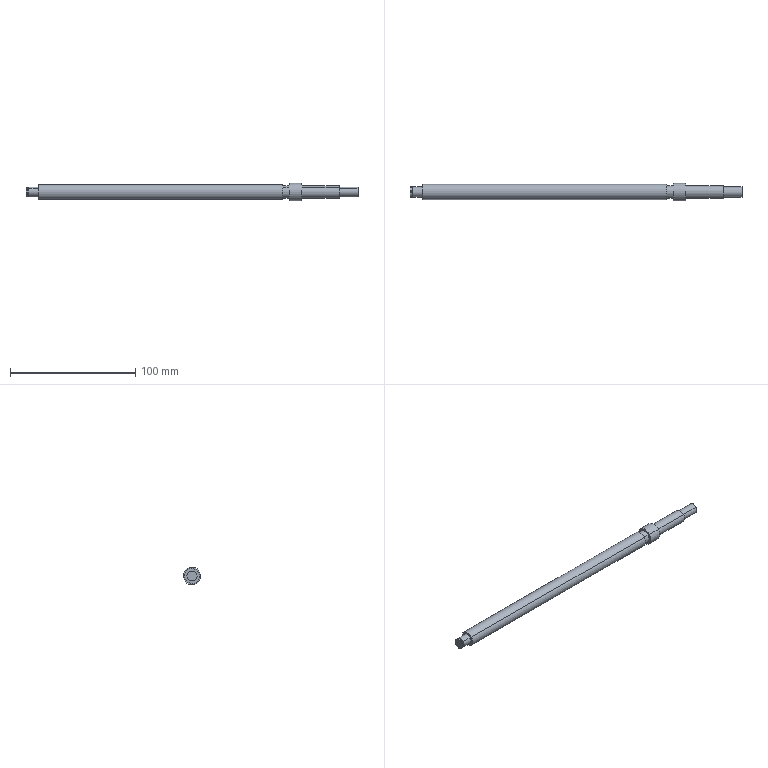Component | SolidWorks | BNK1208-2-ScrewRod-1 | 1 solid | 25 faces | box 265 x 14 x 14 mm | volume 27592 mm3 | cylinder 16 | plane 9 | commonest cylinder face diameters 8 x6 10 x4 7.4 x2 12 x2 14 x2
build123d program:
from build123d import *

# Parameters (mm, degrees)
SKETCH1_R           = 4
BOSS_EXTRUDE1_DEPTH = 15
SKETCH2_R           = 5
BOSS_EXTRUDE2_DEPTH = 30
SKETCH3_R           = 7
BOSS_EXTRUDE3_DEPTH = 10
SKETCH4_R           = 5
BOSS_EXTRUDE4_DEPTH = 5
SKETCH5_R           = 6
BOSS_EXTRUDE5_DEPTH = 195
SKETCH6_R           = 4
BOSS_EXTRUDE6_DEPTH = 10
SKETCH7_W           = 0.3
SKETCH7_H           = 0.9


with BuildPart() as part:
    # Sketch1 → Boss-Extrude1 (new body)
    with BuildSketch(Plane.XY):
        Circle(SKETCH1_R)
    extrude(amount=BOSS_EXTRUDE1_DEPTH)

    # Sketch2 → Boss-Extrude2 (add)
    with BuildSketch(Plane.XY.offset(15)):
        Circle(SKETCH2_R)
    extrude(amount=BOSS_EXTRUDE2_DEPTH)

    # Sketch3 → Boss-Extrude3 (add)
    with BuildSketch(Plane.XY.offset(45)):
        Circle(SKETCH3_R)
    extrude(amount=BOSS_EXTRUDE3_DEPTH)

    # Sketch4 → Boss-Extrude4 (add)
    with BuildSketch(Plane.XY.offset(55)):
        Circle(SKETCH4_R)
    extrude(amount=BOSS_EXTRUDE4_DEPTH)

    # Sketch5 → Boss-Extrude5 (add)
    with BuildSketch(Plane.XY.offset(60)):
        Circle(SKETCH5_R)
    extrude(amount=BOSS_EXTRUDE5_DEPTH)

    # Sketch6 → Boss-Extrude6 (add)
    with BuildSketch(Plane.XY.offset(255)):
        Circle(SKETCH6_R)
    extrude(amount=BOSS_EXTRUDE6_DEPTH)

    # Sketch7 → Cut-Revolve1 (revolve, cut)
    with BuildSketch(Plane(origin=(0, 0, 0), x_dir=(1, 0, 0), z_dir=(0, 1, 0)), mode=Mode.PRIVATE) as cut_revolve1_sk:
        with Locations((-3.85, -263.35)):
            Rectangle(SKETCH7_W, SKETCH7_H)
    revolve(cut_revolve1_sk.sketch.rotate(Axis((0, 0, 255), (0, 0, -1)), 180), axis=Axis((0, 0, 255), (0, 0, -1)), mode=Mode.SUBTRACT)


solid = part.part

# Placed as in the assembly
solid = solid.moved(Location((73.978, 19.945, 3.551), (0, -90, 0)))
STEP:
#1=CARTESIAN_POINT('',(-7.521,0.9056,0.03818));
#2=VERTEX_POINT('',#1);
#3=CARTESIAN_POINT('',(-7.521,0.6649,0.2414));
#4=VERTEX_POINT('',#3);
#5=CARTESIAN_POINT('',(-7.521,0.7853,0.1398));
#6=DIRECTION('',(-1.,0.,0.));
#7=DIRECTION('',(0.,0.764,-0.6453));
#8=AXIS2_PLACEMENT_3D('',#5,#6,#7);
#9=CIRCLE('',#8,0.1575);
#10=EDGE_CURVE('',#2,#4,#9,.T.);
#11=ORIENTED_EDGE('',*,*,#10,.F.);
#12=CARTESIAN_POINT('',(-7.473,0.9056,0.03818));
#13=VERTEX_POINT('',#12);
#14=CARTESIAN_POINT('',(-7.521,0.9056,0.03818));
#15=DIRECTION('',(1.,-0.,-0.));
#16=VECTOR('',#15,39.37);
#17=LINE('',#14,#16);
#18=EDGE_CURVE('',#2,#13,#17,.T.);
#19=ORIENTED_EDGE('',*,*,#18,.T.);
#20=CARTESIAN_POINT('',(-7.473,0.6649,0.2414));
#21=VERTEX_POINT('',#20);
#22=CARTESIAN_POINT('',(-7.473,0.7853,0.1398));
#23=DIRECTION('',(-1.,0.,0.));
#24=DIRECTION('',(0.,0.764,-0.6453));
#25=AXIS2_PLACEMENT_3D('',#22,#23,#24);
#26=CIRCLE('',#25,0.1575);
#27=EDGE_CURVE('',#13,#21,#26,.T.);
#28=ORIENTED_EDGE('',*,*,#27,.T.);
#29=CARTESIAN_POINT('',(-7.521,0.6649,0.2414));
#30=DIRECTION('',(1.,-0.,-0.));
#31=VECTOR('',#30,39.37);
#32=LINE('',#29,#31);
#33=EDGE_CURVE('',#4,#21,#32,.T.);
#34=ORIENTED_EDGE('',*,*,#33,.F.);
#35=EDGE_LOOP('',(#11,#19,#28,#34));
#36=FACE_OUTER_BOUND('',#35,.T.);
#37=CARTESIAN_POINT('',(-7.521,0.7853,0.1398));
#38=DIRECTION('',(1.,-0.,-0.));
#39=DIRECTION('',(0.,-0.764,0.6453));
#40=AXIS2_PLACEMENT_3D('',#37,#38,#39);
#41=CYLINDRICAL_SURFACE('',#40,0.1575);
#42=ADVANCED_FACE('',(#36),#41,.T.);
#43=CARTESIAN_POINT('',(-7.438,0.8965,0.0458));
#44=VERTEX_POINT('',#43);
#45=CARTESIAN_POINT('',(-7.438,0.674,0.2338));
#46=VERTEX_POINT('',#45);
#47=CARTESIAN_POINT('',(-7.438,0.7853,0.1398));
#48=DIRECTION('',(-1.,0.,0.));
#49=DIRECTION('',(0.,0.764,-0.6453));
#50=AXIS2_PLACEMENT_3D('',#47,#48,#49);
#51=CIRCLE('',#50,0.1457);
#52=EDGE_CURVE('',#44,#46,#51,.T.);
#53=ORIENTED_EDGE('',*,*,#52,.T.);
#54=CARTESIAN_POINT('',(-7.473,0.674,0.2338));
#55=VERTEX_POINT('',#54);
#56=CARTESIAN_POINT('',(-7.127,0.674,0.2338));
#57=DIRECTION('',(-1.,0.,0.));
#58=VECTOR('',#57,39.37);
#59=LINE('',#56,#58);
#60=EDGE_CURVE('',#46,#55,#59,.T.);
#61=ORIENTED_EDGE('',*,*,#60,.T.);
#62=CARTESIAN_POINT('',(-7.473,0.8965,0.0458));
#63=VERTEX_POINT('',#62);
#64=CARTESIAN_POINT('',(-7.473,0.7853,0.1398));
#65=DIRECTION('',(-1.,0.,0.));
#66=DIRECTION('',(0.,0.764,-0.6453));
#67=AXIS2_PLACEMENT_3D('',#64,#65,#66);
#68=CIRCLE('',#67,0.1457);
#69=EDGE_CURVE('',#63,#55,#68,.T.);
#70=ORIENTED_EDGE('',*,*,#69,.F.);
#71=CARTESIAN_POINT('',(-7.127,0.8965,0.0458));
#72=DIRECTION('',(-1.,0.,0.));
#73=VECTOR('',#72,39.37);
#74=LINE('',#71,#73);
#75=EDGE_CURVE('',#44,#63,#74,.T.);
#76=ORIENTED_EDGE('',*,*,#75,.F.);
#77=EDGE_LOOP('',(#53,#61,#70,#76));
#78=FACE_OUTER_BOUND('',#77,.T.);
#79=CARTESIAN_POINT('',(-7.127,0.7853,0.1398));
#80=DIRECTION('',(-1.,0.,0.));
#81=DIRECTION('',(0.,0.764,-0.6453));
#82=AXIS2_PLACEMENT_3D('',#79,#80,#81);
#83=CYLINDRICAL_SURFACE('',#82,0.1457);
#84=ADVANCED_FACE('',(#78),#83,.T.);
#85=CARTESIAN_POINT('',(-7.127,0.9657,-0.01263));
#86=VERTEX_POINT('',#85);
#87=CARTESIAN_POINT('',(-7.127,0.6048,0.2922));
#88=VERTEX_POINT('',#87);
#89=CARTESIAN_POINT('',(-7.127,0.7853,0.1398));
#90=DIRECTION('',(-1.,0.,0.));
#91=DIRECTION('',(0.,0.764,-0.6453));
#92=AXIS2_PLACEMENT_3D('',#89,#90,#91);
#93=CIRCLE('',#92,0.2362);
#94=EDGE_CURVE('',#86,#88,#93,.T.);
#95=ORIENTED_EDGE('',*,*,#94,.F.);
#96=CARTESIAN_POINT('',(0.5503,0.9657,-0.01263));
#97=VERTEX_POINT('',#96);
#98=CARTESIAN_POINT('',(-7.127,0.9657,-0.01263));
#99=DIRECTION('',(1.,-0.,-0.));
#100=VECTOR('',#99,39.37);
#101=LINE('',#98,#100);
#102=EDGE_CURVE('',#86,#97,#101,.T.);
#103=ORIENTED_EDGE('',*,*,#102,.T.);
#104=CARTESIAN_POINT('',(0.5503,0.6048,0.2922));
#105=VERTEX_POINT('',#104);
#106=CARTESIAN_POINT('',(0.5503,0.7853,0.1398));
#107=DIRECTION('',(-1.,0.,0.));
#108=DIRECTION('',(0.,0.764,-0.6453));
#109=AXIS2_PLACEMENT_3D('',#106,#107,#108);
#110=CIRCLE('',#109,0.2362);
#111=EDGE_CURVE('',#97,#105,#110,.T.);
#112=ORIENTED_EDGE('',*,*,#111,.T.);
#113=CARTESIAN_POINT('',(-7.127,0.6048,0.2922));
#114=DIRECTION('',(1.,-0.,-0.));
#115=VECTOR('',#114,39.37);
#116=LINE('',#113,#115);
#117=EDGE_CURVE('',#88,#105,#116,.T.);
#118=ORIENTED_EDGE('',*,*,#117,.F.);
#119=EDGE_LOOP('',(#95,#103,#112,#118));
#120=FACE_OUTER_BOUND('',#119,.T.);
#121=CARTESIAN_POINT('',(-7.127,0.7853,0.1398));
#122=DIRECTION('',(1.,-0.,-0.));
#123=DIRECTION('',(0.,-0.764,0.6453));
#124=AXIS2_PLACEMENT_3D('',#121,#122,#123);
#125=CYLINDRICAL_SURFACE('',#124,0.2362);
#126=ADVANCED_FACE('',(#120),#125,.T.);
#127=CARTESIAN_POINT('',(0.5503,0.9356,0.01277));
#128=VERTEX_POINT('',#127);
#129=CARTESIAN_POINT('',(0.5503,0.6349,0.2668));
#130=VERTEX_POINT('',#129);
#131=CARTESIAN_POINT('',(0.5503,0.7853,0.1398));
#132=DIRECTION('',(-1.,0.,0.));
#133=DIRECTION('',(0.,0.764,-0.6453));
#134=AXIS2_PLACEMENT_3D('',#131,#132,#133);
#135=CIRCLE('',#134,0.1969);
#136=EDGE_CURVE('',#128,#130,#135,.T.);
#137=ORIENTED_EDGE('',*,*,#136,.F.);
#138=CARTESIAN_POINT('',(0.7472,0.9356,0.01277));
#139=VERTEX_POINT('',#138);
#140=CARTESIAN_POINT('',(0.5503,0.9356,0.01277));
#141=DIRECTION('',(1.,-0.,-0.));
#142=VECTOR('',#141,39.37);
#143=LINE('',#140,#142);
#144=EDGE_CURVE('',#128,#139,#143,.T.);
#145=ORIENTED_EDGE('',*,*,#144,.T.);
#146=CARTESIAN_POINT('',(0.7472,0.6349,0.2668));
#147=VERTEX_POINT('',#146);
#148=CARTESIAN_POINT('',(0.7472,0.7853,0.1398));
#149=DIRECTION('',(-1.,0.,0.));
#150=DIRECTION('',(0.,0.764,-0.6453));
#151=AXIS2_PLACEMENT_3D('',#148,#149,#150);
#152=CIRCLE('',#151,0.1969);
#153=EDGE_CURVE('',#139,#147,#152,.T.);
#154=ORIENTED_EDGE('',*,*,#153,.T.);
#155=CARTESIAN_POINT('',(0.5503,0.6349,0.2668));
#156=DIRECTION('',(1.,-0.,-0.));
#157=VECTOR('',#156,39.37);
#158=LINE('',#155,#157);
#159=EDGE_CURVE('',#130,#147,#158,.T.);
#160=ORIENTED_EDGE('',*,*,#159,.F.);
#161=EDGE_LOOP('',(#137,#145,#154,#160));
#162=FACE_OUTER_BOUND('',#161,.T.);
#163=CARTESIAN_POINT('',(0.5503,0.7853,0.1398));
#164=DIRECTION('',(1.,-0.,-0.));
#165=DIRECTION('',(0.,-0.764,0.6453));
#166=AXIS2_PLACEMENT_3D('',#163,#164,#165);
#167=CYLINDRICAL_SURFACE('',#166,0.1969);
#168=ADVANCED_FACE('',(#162),#167,.T.);
#169=CARTESIAN_POINT('',(0.7472,0.9958,-0.03804));
#170=VERTEX_POINT('',#169);
#171=CARTESIAN_POINT('',(0.7472,0.5747,0.3176));
#172=VERTEX_POINT('',#171);
#173=CARTESIAN_POINT('',(0.7472,0.7853,0.1398));
#174=DIRECTION('',(-1.,0.,0.));
#175=DIRECTION('',(0.,0.764,-0.6453));
#176=AXIS2_PLACEMENT_3D('',#173,#174,#175);
#177=CIRCLE('',#176,0.2756);
#178=EDGE_CURVE('',#170,#172,#177,.T.);
#179=ORIENTED_EDGE('',*,*,#178,.F.);
#180=CARTESIAN_POINT('',(1.141,0.9958,-0.03804));
#181=VERTEX_POINT('',#180);
#182=CARTESIAN_POINT('',(0.7472,0.9958,-0.03804));
#183=DIRECTION('',(1.,-0.,-0.));
#184=VECTOR('',#183,39.37);
#185=LINE('',#182,#184);
#186=EDGE_CURVE('',#170,#181,#185,.T.);
#187=ORIENTED_EDGE('',*,*,#186,.T.);
#188=CARTESIAN_POINT('',(1.141,0.5747,0.3176));
#189=VERTEX_POINT('',#188);
#190=CARTESIAN_POINT('',(1.141,0.7853,0.1398));
#191=DIRECTION('',(-1.,0.,0.));
#192=DIRECTION('',(0.,0.764,-0.6453));
#193=AXIS2_PLACEMENT_3D('',#190,#191,#192);
#194=CIRCLE('',#193,0.2756);
#195=EDGE_CURVE('',#181,#189,#194,.T.);
#196=ORIENTED_EDGE('',*,*,#195,.T.);
#197=CARTESIAN_POINT('',(0.7472,0.5747,0.3176));
#198=DIRECTION('',(1.,-0.,-0.));
#199=VECTOR('',#198,39.37);
#200=LINE('',#197,#199);
#201=EDGE_CURVE('',#172,#189,#200,.T.);
#202=ORIENTED_EDGE('',*,*,#201,.F.);
#203=EDGE_LOOP('',(#179,#187,#196,#202));
#204=FACE_OUTER_BOUND('',#203,.T.);
#205=CARTESIAN_POINT('',(0.7472,0.7853,0.1398));
#206=DIRECTION('',(1.,-0.,-0.));
#207=DIRECTION('',(0.,-0.764,0.6453));
#208=AXIS2_PLACEMENT_3D('',#205,#206,#207);
#209=CYLINDRICAL_SURFACE('',#208,0.2756);
#210=ADVANCED_FACE('',(#204),#209,.T.);
#211=CARTESIAN_POINT('',(1.141,0.9356,0.01277));
#212=VERTEX_POINT('',#211);
#213=CARTESIAN_POINT('',(1.141,0.6349,0.2668));
#214=VERTEX_POINT('',#213);
#215=CARTESIAN_POINT('',(1.141,0.7853,0.1398));
#216=DIRECTION('',(-1.,0.,0.));
#217=DIRECTION('',(0.,0.764,-0.6453));
#218=AXIS2_PLACEMENT_3D('',#215,#216,#217);
#219=CIRCLE('',#218,0.1969);
#220=EDGE_CURVE('',#212,#214,#219,.T.);
#221=ORIENTED_EDGE('',*,*,#220,.F.);
#222=CARTESIAN_POINT('',(2.322,0.9356,0.01277));
#223=VERTEX_POINT('',#222);
#224=CARTESIAN_POINT('',(1.141,0.9356,0.01277));
#225=DIRECTION('',(1.,-0.,-0.));
#226=VECTOR('',#225,39.37);
#227=LINE('',#224,#226);
#228=EDGE_CURVE('',#212,#223,#227,.T.);
#229=ORIENTED_EDGE('',*,*,#228,.T.);
#230=CARTESIAN_POINT('',(2.322,0.6349,0.2668));
#231=VERTEX_POINT('',#230);
#232=CARTESIAN_POINT('',(2.322,0.7853,0.1398));
#233=DIRECTION('',(-1.,0.,0.));
#234=DIRECTION('',(0.,0.764,-0.6453));
#235=AXIS2_PLACEMENT_3D('',#232,#233,#234);
#236=CIRCLE('',#235,0.1969);
#237=EDGE_CURVE('',#223,#231,#236,.T.);
#238=ORIENTED_EDGE('',*,*,#237,.T.);
#239=CARTESIAN_POINT('',(1.141,0.6349,0.2668));
#240=DIRECTION('',(1.,-0.,-0.));
#241=VECTOR('',#240,39.37);
#242=LINE('',#239,#241);
#243=EDGE_CURVE('',#214,#231,#242,.T.);
#244=ORIENTED_EDGE('',*,*,#243,.F.);
#245=EDGE_LOOP('',(#221,#229,#238,#244));
#246=FACE_OUTER_BOUND('',#245,.T.);
#247=CARTESIAN_POINT('',(1.141,0.7853,0.1398));
#248=DIRECTION('',(1.,-0.,-0.));
#249=DIRECTION('',(0.,-0.764,0.6453));
#250=AXIS2_PLACEMENT_3D('',#247,#248,#249);
#251=CYLINDRICAL_SURFACE('',#250,0.1969);
#252=ADVANCED_FACE('',(#246),#251,.T.);
#253=CARTESIAN_POINT('',(2.322,0.9056,0.03818));
#254=VERTEX_POINT('',#253);
#255=CARTESIAN_POINT('',(2.322,0.6649,0.2414));
#256=VERTEX_POINT('',#255);
#257=CARTESIAN_POINT('',(2.322,0.7853,0.1398));
#258=DIRECTION('',(-1.,0.,0.));
#259=DIRECTION('',(0.,0.764,-0.6453));
#260=AXIS2_PLACEMENT_3D('',#257,#258,#259);
#261=CIRCLE('',#260,0.1575);
#262=EDGE_CURVE('',#254,#256,#261,.T.);
#263=ORIENTED_EDGE('',*,*,#262,.F.);
#264=CARTESIAN_POINT('',(2.913,0.9056,0.03818));
#265=VERTEX_POINT('',#264);
#266=CARTESIAN_POINT('',(2.322,0.9056,0.03818));
#267=DIRECTION('',(1.,-0.,-0.));
#268=VECTOR('',#267,39.37);
#269=LINE('',#266,#268);
#270=EDGE_CURVE('',#254,#265,#269,.T.);
#271=ORIENTED_EDGE('',*,*,#270,.T.);
#272=CARTESIAN_POINT('',(2.913,0.6649,0.2414));
#273=VERTEX_POINT('',#272);
#274=CARTESIAN_POINT('',(2.913,0.7853,0.1398));
#275=DIRECTION('',(-1.,0.,0.));
#276=DIRECTION('',(0.,0.764,-0.6453));
#277=AXIS2_PLACEMENT_3D('',#274,#275,#276);
#278=CIRCLE('',#277,0.1575);
#279=EDGE_CURVE('',#265,#273,#278,.T.);
#280=ORIENTED_EDGE('',*,*,#279,.T.);
#281=CARTESIAN_POINT('',(2.322,0.6649,0.2414));
#282=DIRECTION('',(1.,-0.,-0.));
#283=VECTOR('',#282,39.37);
#284=LINE('',#281,#283);
#285=EDGE_CURVE('',#256,#273,#284,.T.);
#286=ORIENTED_EDGE('',*,*,#285,.F.);
#287=EDGE_LOOP('',(#263,#271,#280,#286));
#288=FACE_OUTER_BOUND('',#287,.T.);
#289=CARTESIAN_POINT('',(2.322,0.7853,0.1398));
#290=DIRECTION('',(1.,-0.,-0.));
#291=DIRECTION('',(0.,-0.764,0.6453));
#292=AXIS2_PLACEMENT_3D('',#289,#290,#291);
#293=CYLINDRICAL_SURFACE('',#292,0.1575);
#294=ADVANCED_FACE('',(#288),#293,.T.);
#295=CARTESIAN_POINT('',(-7.438,0.9056,0.03818));
#296=VERTEX_POINT('',#295);
#297=CARTESIAN_POINT('',(-7.438,0.6649,0.2414));
#298=VERTEX_POINT('',#297);
#299=CARTESIAN_POINT('',(-7.438,0.7853,0.1398));
#300=DIRECTION('',(-1.,0.,0.));
#301=DIRECTION('',(0.,0.764,-0.6453));
#302=AXIS2_PLACEMENT_3D('',#299,#300,#301);
#303=CIRCLE('',#302,0.1575);
#304=EDGE_CURVE('',#296,#298,#303,.T.);
#305=ORIENTED_EDGE('',*,*,#304,.F.);
#306=CARTESIAN_POINT('',(-7.127,0.9056,0.03818));
#307=VERTEX_POINT('',#306);
#308=CARTESIAN_POINT('',(-7.521,0.9056,0.03818));
#309=DIRECTION('',(1.,-0.,-0.));
#310=VECTOR('',#309,39.37);
#311=LINE('',#308,#310);
#312=EDGE_CURVE('',#296,#307,#311,.T.);
#313=ORIENTED_EDGE('',*,*,#312,.T.);
#314=CARTESIAN_POINT('',(-7.127,0.6649,0.2414));
#315=VERTEX_POINT('',#314);
#316=CARTESIAN_POINT('',(-7.127,0.7853,0.1398));
#317=DIRECTION('',(-1.,0.,0.));
#318=DIRECTION('',(0.,0.764,-0.6453));
#319=AXIS2_PLACEMENT_3D('',#316,#317,#318);
#320=CIRCLE('',#319,0.1575);
#321=EDGE_CURVE('',#307,#315,#320,.T.);
#322=ORIENTED_EDGE('',*,*,#321,.T.);
#323=CARTESIAN_POINT('',(-7.521,0.6649,0.2414));
#324=DIRECTION('',(1.,-0.,-0.));
#325=VECTOR('',#324,39.37);
#326=LINE('',#323,#325);
#327=EDGE_CURVE('',#298,#315,#326,.T.);
#328=ORIENTED_EDGE('',*,*,#327,.F.);
#329=EDGE_LOOP('',(#305,#313,#322,#328));
#330=FACE_OUTER_BOUND('',#329,.T.);
#331=CARTESIAN_POINT('',(-7.521,0.7853,0.1398));
#332=DIRECTION('',(1.,-0.,-0.));
#333=DIRECTION('',(0.,-0.764,0.6453));
#334=AXIS2_PLACEMENT_3D('',#331,#332,#333);
#335=CYLINDRICAL_SURFACE('',#334,0.1575);
#336=ADVANCED_FACE('',(#330),#335,.T.);
#337=ORIENTED_EDGE('',*,*,#312,.F.);
#338=CARTESIAN_POINT('',(-7.438,0.7853,0.1398));
#339=DIRECTION('',(-1.,0.,0.));
#340=DIRECTION('',(0.,0.764,-0.6453));
#341=AXIS2_PLACEMENT_3D('',#338,#339,#340);
#342=CIRCLE('',#341,0.1575);
#343=EDGE_CURVE('',#298,#296,#342,.T.);
#344=ORIENTED_EDGE('',*,*,#343,.F.);
#345=ORIENTED_EDGE('',*,*,#327,.T.);
#346=CARTESIAN_POINT('',(-7.127,0.7853,0.1398));
#347=DIRECTION('',(-1.,0.,0.));
#348=DIRECTION('',(0.,0.764,-0.6453));
#349=AXIS2_PLACEMENT_3D('',#346,#347,#348);
#350=CIRCLE('',#349,0.1575);
#351=EDGE_CURVE('',#315,#307,#350,.T.);
#352=ORIENTED_EDGE('',*,*,#351,.T.);
#353=EDGE_LOOP('',(#337,#344,#345,#352));
#354=FACE_OUTER_BOUND('',#353,.T.);
#355=CARTESIAN_POINT('',(-7.521,0.7853,0.1398));
#356=DIRECTION('',(1.,-0.,-0.));
#357=DIRECTION('',(0.,-0.764,0.6453));
#358=AXIS2_PLACEMENT_3D('',#355,#356,#357);
#359=CYLINDRICAL_SURFACE('',#358,0.1575);
#360=ADVANCED_FACE('',(#354),#359,.T.);
#361=CARTESIAN_POINT('',(-7.127,0.7853,0.1398));
#362=DIRECTION('',(-1.,0.,0.));
#363=DIRECTION('',(0.,0.764,-0.6453));
#364=AXIS2_PLACEMENT_3D('',#361,#362,#363);
#365=CIRCLE('',#364,0.2362);
#366=EDGE_CURVE('',#88,#86,#365,.T.);
#367=ORIENTED_EDGE('',*,*,#366,.T.);
#368=ORIENTED_EDGE('',*,*,#94,.T.);
#369=EDGE_LOOP('',(#367,#368));
#370=FACE_OUTER_BOUND('',#369,.T.);
#371=ORIENTED_EDGE('',*,*,#351,.F.);
#372=ORIENTED_EDGE('',*,*,#321,.F.);
#373=EDGE_LOOP('',(#371,#372));
#374=FACE_BOUND('',#373,.T.);
#375=CARTESIAN_POINT('',(-7.127,0.7853,0.1398));
#376=DIRECTION('',(-1.,0.,0.));
#377=DIRECTION('',(-0.,0.764,-0.6453));
#378=AXIS2_PLACEMENT_3D('',#375,#376,#377);
#379=PLANE('',#378);
#380=ADVANCED_FACE('',(#370,#374),#379,.T.);
#381=CARTESIAN_POINT('',(0.7472,0.7853,0.1398));
#382=DIRECTION('',(-1.,0.,0.));
#383=DIRECTION('',(0.,0.764,-0.6453));
#384=AXIS2_PLACEMENT_3D('',#381,#382,#383);
#385=CIRCLE('',#384,0.2756);
#386=EDGE_CURVE('',#172,#170,#385,.T.);
#387=ORIENTED_EDGE('',*,*,#386,.T.);
#388=ORIENTED_EDGE('',*,*,#178,.T.);
#389=EDGE_LOOP('',(#387,#388));
#390=FACE_OUTER_BOUND('',#389,.T.);
#391=CARTESIAN_POINT('',(0.7472,0.7853,0.1398));
#392=DIRECTION('',(-1.,0.,0.));
#393=DIRECTION('',(0.,0.764,-0.6453));
#394=AXIS2_PLACEMENT_3D('',#391,#392,#393);
#395=CIRCLE('',#394,0.1969);
#396=EDGE_CURVE('',#147,#139,#395,.T.);
#397=ORIENTED_EDGE('',*,*,#396,.F.);
#398=ORIENTED_EDGE('',*,*,#153,.F.);
#399=EDGE_LOOP('',(#397,#398));
#400=FACE_BOUND('',#399,.T.);
#401=CARTESIAN_POINT('',(0.7472,0.7853,0.1398));
#402=DIRECTION('',(-1.,0.,0.));
#403=DIRECTION('',(-0.,0.764,-0.6453));
#404=AXIS2_PLACEMENT_3D('',#401,#402,#403);
#405=PLANE('',#404);
#406=ADVANCED_FACE('',(#390,#400),#405,.T.);
#407=ORIENTED_EDGE('',*,*,#270,.F.);
#408=CARTESIAN_POINT('',(2.322,0.7853,0.1398));
#409=DIRECTION('',(-1.,0.,0.));
#410=DIRECTION('',(0.,0.764,-0.6453));
#411=AXIS2_PLACEMENT_3D('',#408,#409,#410);
#412=CIRCLE('',#411,0.1575);
#413=EDGE_CURVE('',#256,#254,#412,.T.);
#414=ORIENTED_EDGE('',*,*,#413,.F.);
#415=ORIENTED_EDGE('',*,*,#285,.T.);
#416=CARTESIAN_POINT('',(2.913,0.7853,0.1398));
#417=DIRECTION('',(-1.,0.,0.));
#418=DIRECTION('',(0.,0.764,-0.6453));
#419=AXIS2_PLACEMENT_3D('',#416,#417,#418);
#420=CIRCLE('',#419,0.1575);
#421=EDGE_CURVE('',#273,#265,#420,.T.);
#422=ORIENTED_EDGE('',*,*,#421,.T.);
#423=EDGE_LOOP('',(#407,#414,#415,#422));
#424=FACE_OUTER_BOUND('',#423,.T.);
#425=CARTESIAN_POINT('',(2.322,0.7853,0.1398));
#426=DIRECTION('',(1.,-0.,-0.));
#427=DIRECTION('',(0.,-0.764,0.6453));
#428=AXIS2_PLACEMENT_3D('',#425,#426,#427);
#429=CYLINDRICAL_SURFACE('',#428,0.1575);
#430=ADVANCED_FACE('',(#424),#429,.T.);
#431=ORIENTED_EDGE('',*,*,#421,.F.);
#432=ORIENTED_EDGE('',*,*,#279,.F.);
#433=EDGE_LOOP('',(#431,#432));
#434=FACE_OUTER_BOUND('',#433,.T.);
#435=CARTESIAN_POINT('',(2.913,0.7853,0.1398));
#436=DIRECTION('',(-1.,0.,0.));
#437=DIRECTION('',(-0.,0.764,-0.6453));
#438=AXIS2_PLACEMENT_3D('',#435,#436,#437);
#439=PLANE('',#438);
#440=ADVANCED_FACE('',(#434),#439,.F.);
#441=CARTESIAN_POINT('',(2.322,0.7853,0.1398));
#442=DIRECTION('',(-1.,0.,0.));
#443=DIRECTION('',(0.,0.764,-0.6453));
#444=AXIS2_PLACEMENT_3D('',#441,#442,#443);
#445=CIRCLE('',#444,0.1969);
#446=EDGE_CURVE('',#231,#223,#445,.T.);
#447=ORIENTED_EDGE('',*,*,#446,.F.);
#448=ORIENTED_EDGE('',*,*,#237,.F.);
#449=EDGE_LOOP('',(#447,#448));
#450=FACE_OUTER_BOUND('',#449,.T.);
#451=ORIENTED_EDGE('',*,*,#413,.T.);
#452=ORIENTED_EDGE('',*,*,#262,.T.);
#453=EDGE_LOOP('',(#451,#452));
#454=FACE_BOUND('',#453,.T.);
#455=CARTESIAN_POINT('',(2.322,0.7853,0.1398));
#456=DIRECTION('',(-1.,0.,0.));
#457=DIRECTION('',(-0.,0.764,-0.6453));
#458=AXIS2_PLACEMENT_3D('',#455,#456,#457);
#459=PLANE('',#458);
#460=ADVANCED_FACE('',(#450,#454),#459,.F.);
#461=ORIENTED_EDGE('',*,*,#228,.F.);
#462=CARTESIAN_POINT('',(1.141,0.7853,0.1398));
#463=DIRECTION('',(-1.,0.,0.));
#464=DIRECTION('',(0.,0.764,-0.6453));
#465=AXIS2_PLACEMENT_3D('',#462,#463,#464);
#466=CIRCLE('',#465,0.1969);
#467=EDGE_CURVE('',#214,#212,#466,.T.);
#468=ORIENTED_EDGE('',*,*,#467,.F.);
#469=ORIENTED_EDGE('',*,*,#243,.T.);
#470=ORIENTED_EDGE('',*,*,#446,.T.);
#471=EDGE_LOOP('',(#461,#468,#469,#470));
#472=FACE_OUTER_BOUND('',#471,.T.);
#473=CARTESIAN_POINT('',(1.141,0.7853,0.1398));
#474=DIRECTION('',(1.,-0.,-0.));
#475=DIRECTION('',(0.,-0.764,0.6453));
#476=AXIS2_PLACEMENT_3D('',#473,#474,#475);
#477=CYLINDRICAL_SURFACE('',#476,0.1969);
#478=ADVANCED_FACE('',(#472),#477,.T.);
#479=CARTESIAN_POINT('',(1.141,0.7853,0.1398));
#480=DIRECTION('',(-1.,0.,0.));
#481=DIRECTION('',(0.,0.764,-0.6453));
#482=AXIS2_PLACEMENT_3D('',#479,#480,#481);
#483=CIRCLE('',#482,0.2756);
#484=EDGE_CURVE('',#189,#181,#483,.T.);
#485=ORIENTED_EDGE('',*,*,#484,.F.);
#486=ORIENTED_EDGE('',*,*,#195,.F.);
#487=EDGE_LOOP('',(#485,#486));
#488=FACE_OUTER_BOUND('',#487,.T.);
#489=ORIENTED_EDGE('',*,*,#467,.T.);
#490=ORIENTED_EDGE('',*,*,#220,.T.);
#491=EDGE_LOOP('',(#489,#490));
#492=FACE_BOUND('',#491,.T.);
#493=CARTESIAN_POINT('',(1.141,0.7853,0.1398));
#494=DIRECTION('',(-1.,0.,0.));
#495=DIRECTION('',(-0.,0.764,-0.6453));
#496=AXIS2_PLACEMENT_3D('',#493,#494,#495);
#497=PLANE('',#496);
#498=ADVANCED_FACE('',(#488,#492),#497,.F.);
#499=ORIENTED_EDGE('',*,*,#186,.F.);
#500=ORIENTED_EDGE('',*,*,#386,.F.);
#501=ORIENTED_EDGE('',*,*,#201,.T.);
#502=ORIENTED_EDGE('',*,*,#484,.T.);
#503=EDGE_LOOP('',(#499,#500,#501,#502));
#504=FACE_OUTER_BOUND('',#503,.T.);
#505=CARTESIAN_POINT('',(0.7472,0.7853,0.1398));
#506=DIRECTION('',(1.,-0.,-0.));
#507=DIRECTION('',(0.,-0.764,0.6453));
#508=AXIS2_PLACEMENT_3D('',#505,#506,#507);
#509=CYLINDRICAL_SURFACE('',#508,0.2756);
#510=ADVANCED_FACE('',(#504),#509,.T.);
#511=ORIENTED_EDGE('',*,*,#144,.F.);
#512=CARTESIAN_POINT('',(0.5503,0.7853,0.1398));
#513=DIRECTION('',(-1.,0.,0.));
#514=DIRECTION('',(0.,0.764,-0.6453));
#515=AXIS2_PLACEMENT_3D('',#512,#513,#514);
#516=CIRCLE('',#515,0.1969);
#517=EDGE_CURVE('',#130,#128,#516,.T.);
#518=ORIENTED_EDGE('',*,*,#517,.F.);
#519=ORIENTED_EDGE('',*,*,#159,.T.);
#520=ORIENTED_EDGE('',*,*,#396,.T.);
#521=EDGE_LOOP('',(#511,#518,#519,#520));
#522=FACE_OUTER_BOUND('',#521,.T.);
#523=CARTESIAN_POINT('',(0.5503,0.7853,0.1398));
#524=DIRECTION('',(1.,-0.,-0.));
#525=DIRECTION('',(0.,-0.764,0.6453));
#526=AXIS2_PLACEMENT_3D('',#523,#524,#525);
#527=CYLINDRICAL_SURFACE('',#526,0.1969);
#528=ADVANCED_FACE('',(#522),#527,.T.);
#529=CARTESIAN_POINT('',(0.5503,0.7853,0.1398));
#530=DIRECTION('',(-1.,0.,0.));
#531=DIRECTION('',(0.,0.764,-0.6453));
#532=AXIS2_PLACEMENT_3D('',#529,#530,#531);
#533=CIRCLE('',#532,0.2362);
#534=EDGE_CURVE('',#105,#97,#533,.T.);
#535=ORIENTED_EDGE('',*,*,#534,.F.);
#536=ORIENTED_EDGE('',*,*,#111,.F.);
#537=EDGE_LOOP('',(#535,#536));
#538=FACE_OUTER_BOUND('',#537,.T.);
#539=ORIENTED_EDGE('',*,*,#517,.T.);
#540=ORIENTED_EDGE('',*,*,#136,.T.);
#541=EDGE_LOOP('',(#539,#540));
#542=FACE_BOUND('',#541,.T.);
#543=CARTESIAN_POINT('',(0.5503,0.7853,0.1398));
#544=DIRECTION('',(-1.,0.,0.));
#545=DIRECTION('',(-0.,0.764,-0.6453));
#546=AXIS2_PLACEMENT_3D('',#543,#544,#545);
#547=PLANE('',#546);
#548=ADVANCED_FACE('',(#538,#542),#547,.F.);
#549=ORIENTED_EDGE('',*,*,#102,.F.);
#550=ORIENTED_EDGE('',*,*,#366,.F.);
#551=ORIENTED_EDGE('',*,*,#117,.T.);
#552=ORIENTED_EDGE('',*,*,#534,.T.);
#553=EDGE_LOOP('',(#549,#550,#551,#552));
#554=FACE_OUTER_BOUND('',#553,.T.);
#555=CARTESIAN_POINT('',(-7.127,0.7853,0.1398));
#556=DIRECTION('',(1.,-0.,-0.));
#557=DIRECTION('',(0.,-0.764,0.6453));
#558=AXIS2_PLACEMENT_3D('',#555,#556,#557);
#559=CYLINDRICAL_SURFACE('',#558,0.2362);
#560=ADVANCED_FACE('',(#554),#559,.T.);
#561=ORIENTED_EDGE('',*,*,#343,.T.);
#562=ORIENTED_EDGE('',*,*,#304,.T.);
#563=EDGE_LOOP('',(#561,#562));
#564=FACE_OUTER_BOUND('',#563,.T.);
#565=ORIENTED_EDGE('',*,*,#52,.F.);
#566=CARTESIAN_POINT('',(-7.438,0.7853,0.1398));
#567=DIRECTION('',(-1.,0.,0.));
#568=DIRECTION('',(0.,0.764,-0.6453));
#569=AXIS2_PLACEMENT_3D('',#566,#567,#568);
#570=CIRCLE('',#569,0.1457);
#571=EDGE_CURVE('',#46,#44,#570,.T.);
#572=ORIENTED_EDGE('',*,*,#571,.F.);
#573=EDGE_LOOP('',(#565,#572));
#574=FACE_BOUND('',#573,.T.);
#575=CARTESIAN_POINT('',(-7.438,0.6649,0.2414));
#576=DIRECTION('',(-1.,0.,0.));
#577=DIRECTION('',(-0.,0.764,-0.6453));
#578=AXIS2_PLACEMENT_3D('',#575,#576,#577);
#579=PLANE('',#578);
#580=ADVANCED_FACE('',(#564,#574),#579,.T.);
#581=ORIENTED_EDGE('',*,*,#60,.F.);
#582=ORIENTED_EDGE('',*,*,#571,.T.);
#583=ORIENTED_EDGE('',*,*,#75,.T.);
#584=CARTESIAN_POINT('',(-7.473,0.7853,0.1398));
#585=DIRECTION('',(-1.,0.,0.));
#586=DIRECTION('',(0.,0.764,-0.6453));
#587=AXIS2_PLACEMENT_3D('',#584,#585,#586);
#588=CIRCLE('',#587,0.1457);
#589=EDGE_CURVE('',#55,#63,#588,.T.);
#590=ORIENTED_EDGE('',*,*,#589,.F.);
#591=EDGE_LOOP('',(#581,#582,#583,#590));
#592=FACE_OUTER_BOUND('',#591,.T.);
#593=CARTESIAN_POINT('',(-7.127,0.7853,0.1398));
#594=DIRECTION('',(-1.,0.,0.));
#595=DIRECTION('',(0.,0.764,-0.6453));
#596=AXIS2_PLACEMENT_3D('',#593,#594,#595);
#597=CYLINDRICAL_SURFACE('',#596,0.1457);
#598=ADVANCED_FACE('',(#592),#597,.T.);
#599=ORIENTED_EDGE('',*,*,#69,.T.);
#600=ORIENTED_EDGE('',*,*,#589,.T.);
#601=EDGE_LOOP('',(#599,#600));
#602=FACE_BOUND('',#601,.T.);
#603=CARTESIAN_POINT('',(-7.473,0.7853,0.1398));
#604=DIRECTION('',(-1.,0.,0.));
#605=DIRECTION('',(0.,0.764,-0.6453));
#606=AXIS2_PLACEMENT_3D('',#603,#604,#605);
#607=CIRCLE('',#606,0.1575);
#608=EDGE_CURVE('',#21,#13,#607,.T.);
#609=ORIENTED_EDGE('',*,*,#608,.F.);
#610=ORIENTED_EDGE('',*,*,#27,.F.);
#611=EDGE_LOOP('',(#609,#610));
#612=FACE_OUTER_BOUND('',#611,.T.);
#613=CARTESIAN_POINT('',(-7.473,0.6649,0.2414));
#614=DIRECTION('',(1.,-0.,-0.));
#615=DIRECTION('',(0.,-0.764,0.6453));
#616=AXIS2_PLACEMENT_3D('',#613,#614,#615);
#617=PLANE('',#616);
#618=ADVANCED_FACE('',(#602,#612),#617,.T.);
#619=CARTESIAN_POINT('',(-7.521,0.7853,0.1398));
#620=DIRECTION('',(-1.,0.,0.));
#621=DIRECTION('',(0.,0.764,-0.6453));
#622=AXIS2_PLACEMENT_3D('',#619,#620,#621);
#623=CIRCLE('',#622,0.1575);
#624=EDGE_CURVE('',#4,#2,#623,.T.);
#625=ORIENTED_EDGE('',*,*,#624,.T.);
#626=ORIENTED_EDGE('',*,*,#10,.T.);
#627=EDGE_LOOP('',(#625,#626));
#628=FACE_OUTER_BOUND('',#627,.T.);
#629=CARTESIAN_POINT('',(-7.521,0.7853,0.1398));
#630=DIRECTION('',(-1.,0.,0.));
#631=DIRECTION('',(-0.,0.764,-0.6453));
#632=AXIS2_PLACEMENT_3D('',#629,#630,#631);
#633=PLANE('',#632);
#634=ADVANCED_FACE('',(#628),#633,.T.);
#635=ORIENTED_EDGE('',*,*,#18,.F.);
#636=ORIENTED_EDGE('',*,*,#624,.F.);
#637=ORIENTED_EDGE('',*,*,#33,.T.);
#638=ORIENTED_EDGE('',*,*,#608,.T.);
#639=EDGE_LOOP('',(#635,#636,#637,#638));
#640=FACE_OUTER_BOUND('',#639,.T.);
#641=CARTESIAN_POINT('',(-7.521,0.7853,0.1398));
#642=DIRECTION('',(1.,-0.,-0.));
#643=DIRECTION('',(0.,-0.764,0.6453));
#644=AXIS2_PLACEMENT_3D('',#641,#642,#643);
#645=CYLINDRICAL_SURFACE('',#644,0.1575);
#646=ADVANCED_FACE('',(#640),#645,.T.);
#647=CLOSED_SHELL('',(#42,#84,#126,#168,#210,#252,#294,#336,#360,#380,#406,#430,#440,#460,#478,#498,#510,#528,#548,#560,#580,#598,#618,#634,#646));
#648=MANIFOLD_SOLID_BREP('',#647);
#649=CARTESIAN_POINT('',(0.,0.,0.));
#650=DIRECTION('',(0.,0.,1.));
#651=DIRECTION('',(1.,0.,0.));
#652=AXIS2_PLACEMENT_3D('',#649,#650,#651);
#653=(LENGTH_UNIT()NAMED_UNIT(*)SI_UNIT($,.METRE.));
#654=LENGTH_MEASURE_WITH_UNIT(LENGTH_MEASURE(0.0254),#653);
#655=DIMENSIONAL_EXPONENTS(1.,0.,0.,0.,0.,0.,0.);
#656=(CONVERSION_BASED_UNIT('',#654)LENGTH_UNIT()NAMED_UNIT(#655));
#657=UNCERTAINTY_MEASURE_WITH_UNIT(LENGTH_MEASURE(0.00001),#656,'','');
#658=(NAMED_UNIT(*)PLANE_ANGLE_UNIT()SI_UNIT($,.RADIAN.));
#659=(NAMED_UNIT(*)SI_UNIT($,.STERADIAN.)SOLID_ANGLE_UNIT());
#660=(GEOMETRIC_REPRESENTATION_CONTEXT(3)GLOBAL_UNCERTAINTY_ASSIGNED_CONTEXT((#657))GLOBAL_UNIT_ASSIGNED_CONTEXT((#656,#658,#659))REPRESENTATION_CONTEXT('',''));
#661=ADVANCED_BREP_SHAPE_REPRESENTATION('',(#648,#652),#660);
#662=COLOUR_RGB('',0.7922,0.8196,0.9333);
#663=FILL_AREA_STYLE_COLOUR('',#662);
#664=FILL_AREA_STYLE('',(#663));
#665=SURFACE_STYLE_FILL_AREA(#664);
#666=SURFACE_SIDE_STYLE('',(#665));
#667=SURFACE_STYLE_USAGE(.BOTH.,#666);
#668=PRESENTATION_STYLE_ASSIGNMENT((#667));
#669=STYLED_ITEM('',(#668),#648);
#670=(LENGTH_UNIT()NAMED_UNIT(*)SI_UNIT($,.METRE.));
#671=LENGTH_MEASURE_WITH_UNIT(LENGTH_MEASURE(0.0254),#670);
#672=DIMENSIONAL_EXPONENTS(1.,0.,0.,0.,0.,0.,0.);
#673=(CONVERSION_BASED_UNIT('',#671)LENGTH_UNIT()NAMED_UNIT(#672));
#674=UNCERTAINTY_MEASURE_WITH_UNIT(LENGTH_MEASURE(0.00001),#673,'','');
#675=(NAMED_UNIT(*)PLANE_ANGLE_UNIT()SI_UNIT($,.RADIAN.));
#676=(NAMED_UNIT(*)SI_UNIT($,.STERADIAN.)SOLID_ANGLE_UNIT());
#677=(GEOMETRIC_REPRESENTATION_CONTEXT(3)GLOBAL_UNCERTAINTY_ASSIGNED_CONTEXT((#674))GLOBAL_UNIT_ASSIGNED_CONTEXT((#673,#675,#676))REPRESENTATION_CONTEXT('',''));
#678=MECHANICAL_DESIGN_GEOMETRIC_PRESENTATION_REPRESENTATION('',(#669),#677);
#679=PRESENTATION_LAYER_ASSIGNMENT('','',(#669));